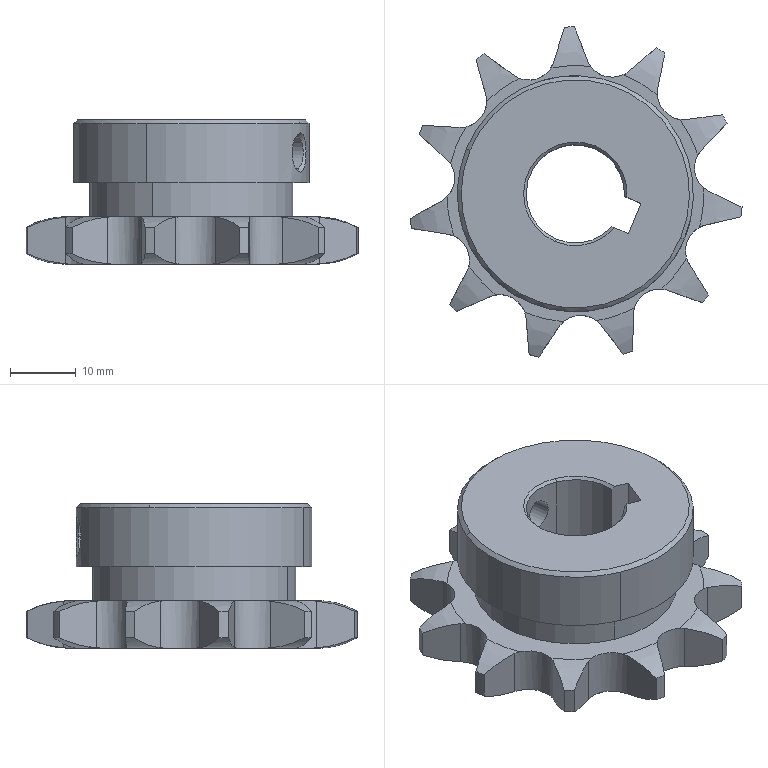Component | SolidWorks | 170423A4-ConveyorSynchronousPulleyAssembly-1_170423A4-VLF02-40-11-D15-1 | 1 solid | 101 faces | volume 19059 mm3 | cylinder 36 | plane 29 | spline 24 | cone 12 | commonest cylinder face diameters 8.041 x14 51 x11 4.917 x4 15 x3 36 x2 31 x2